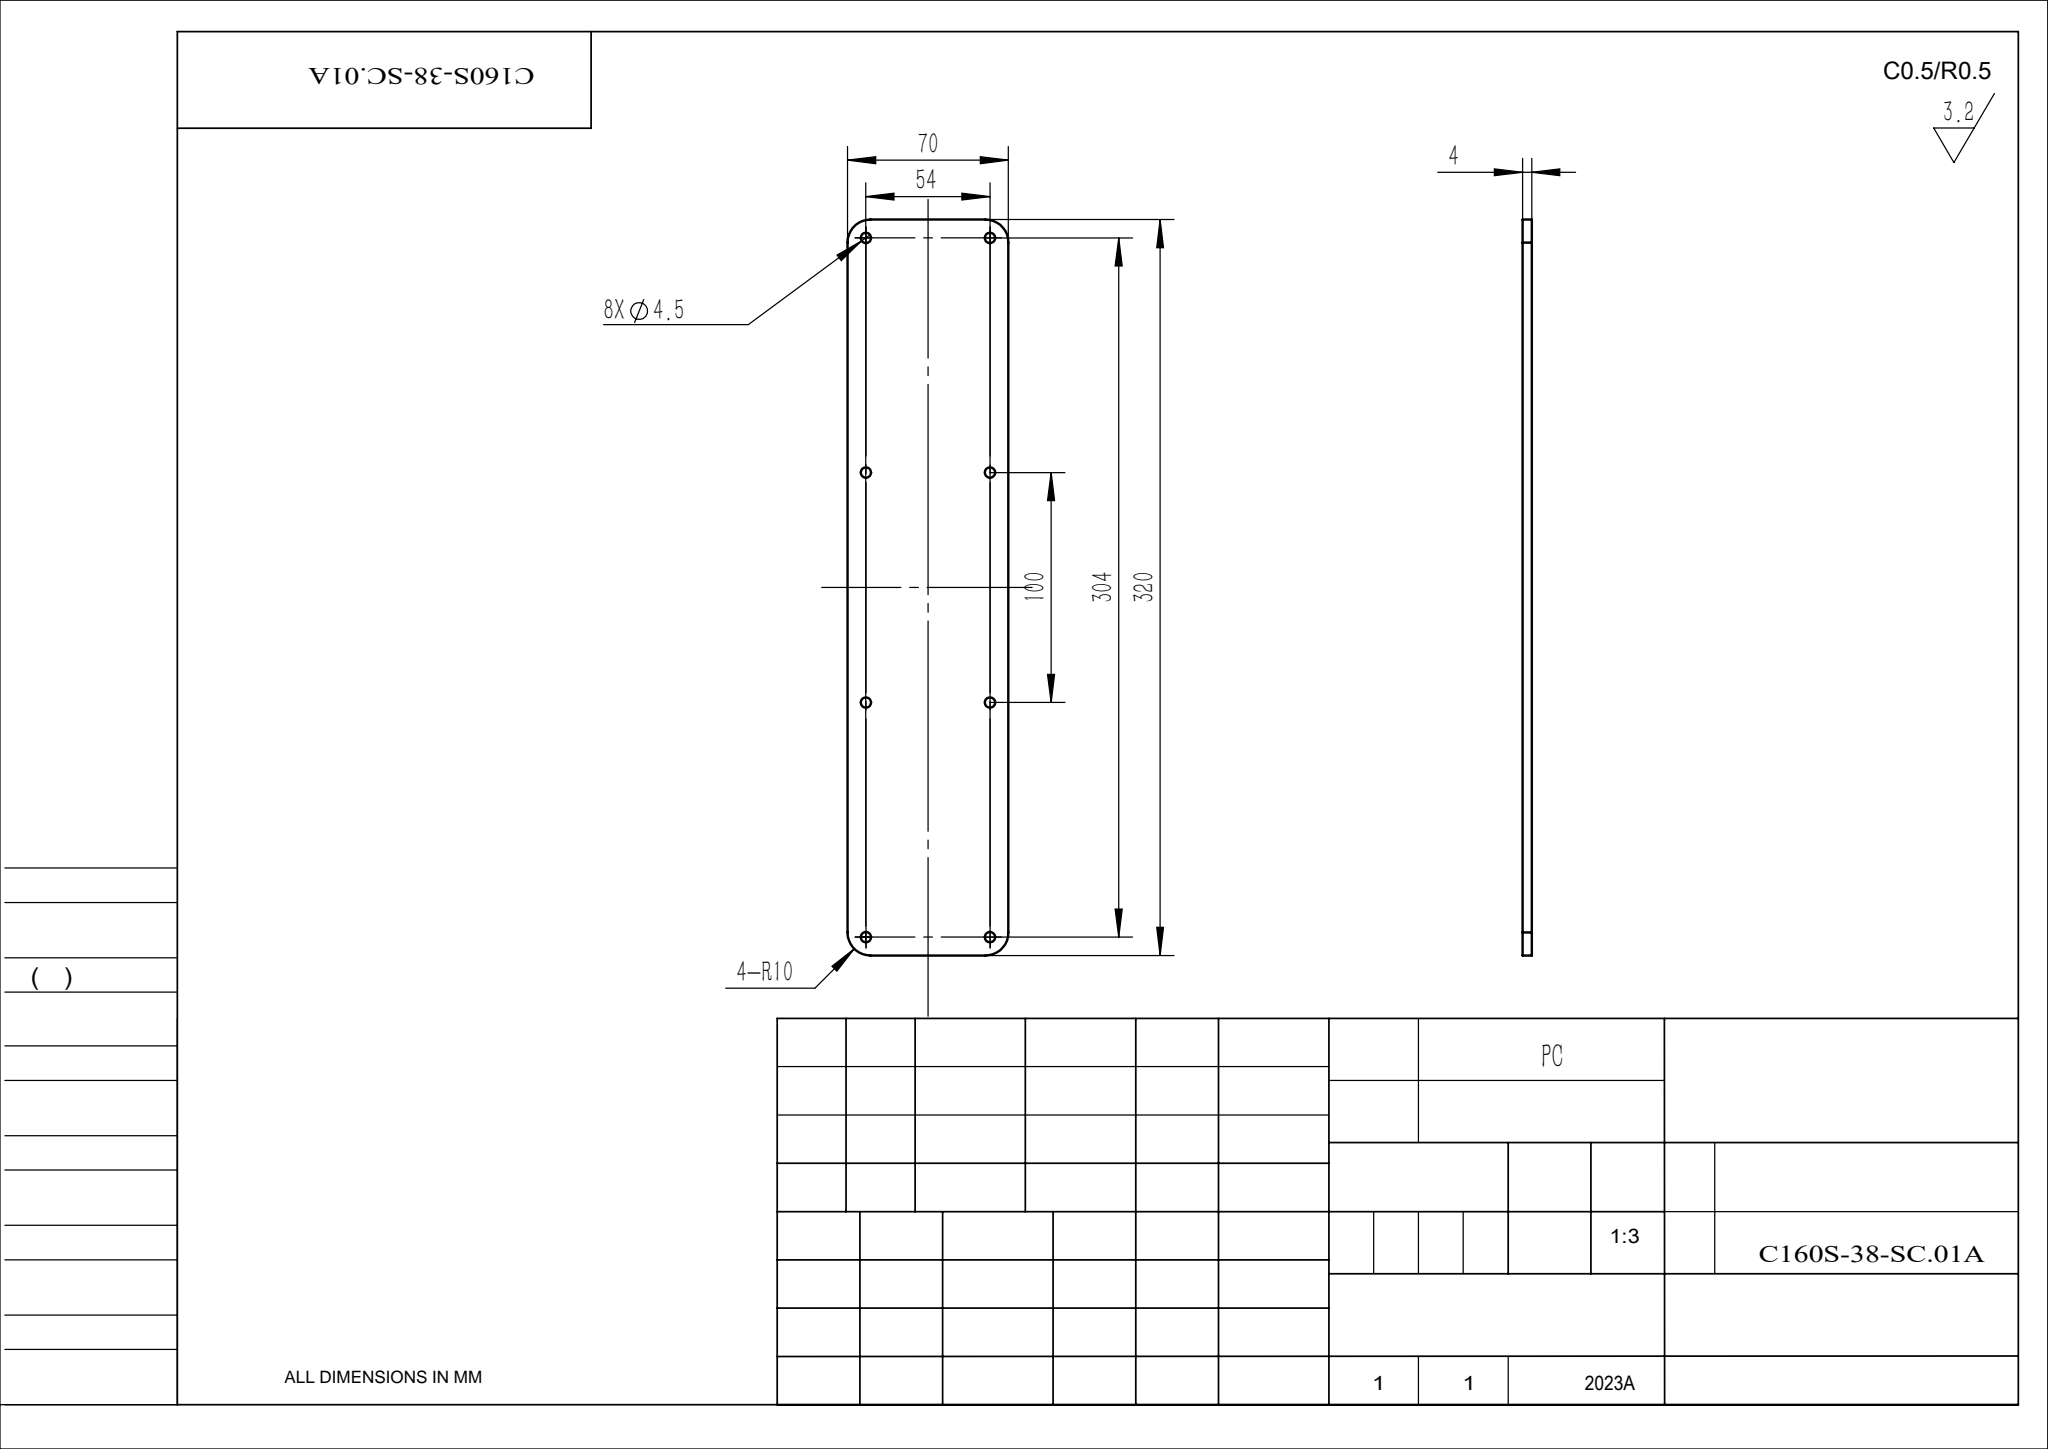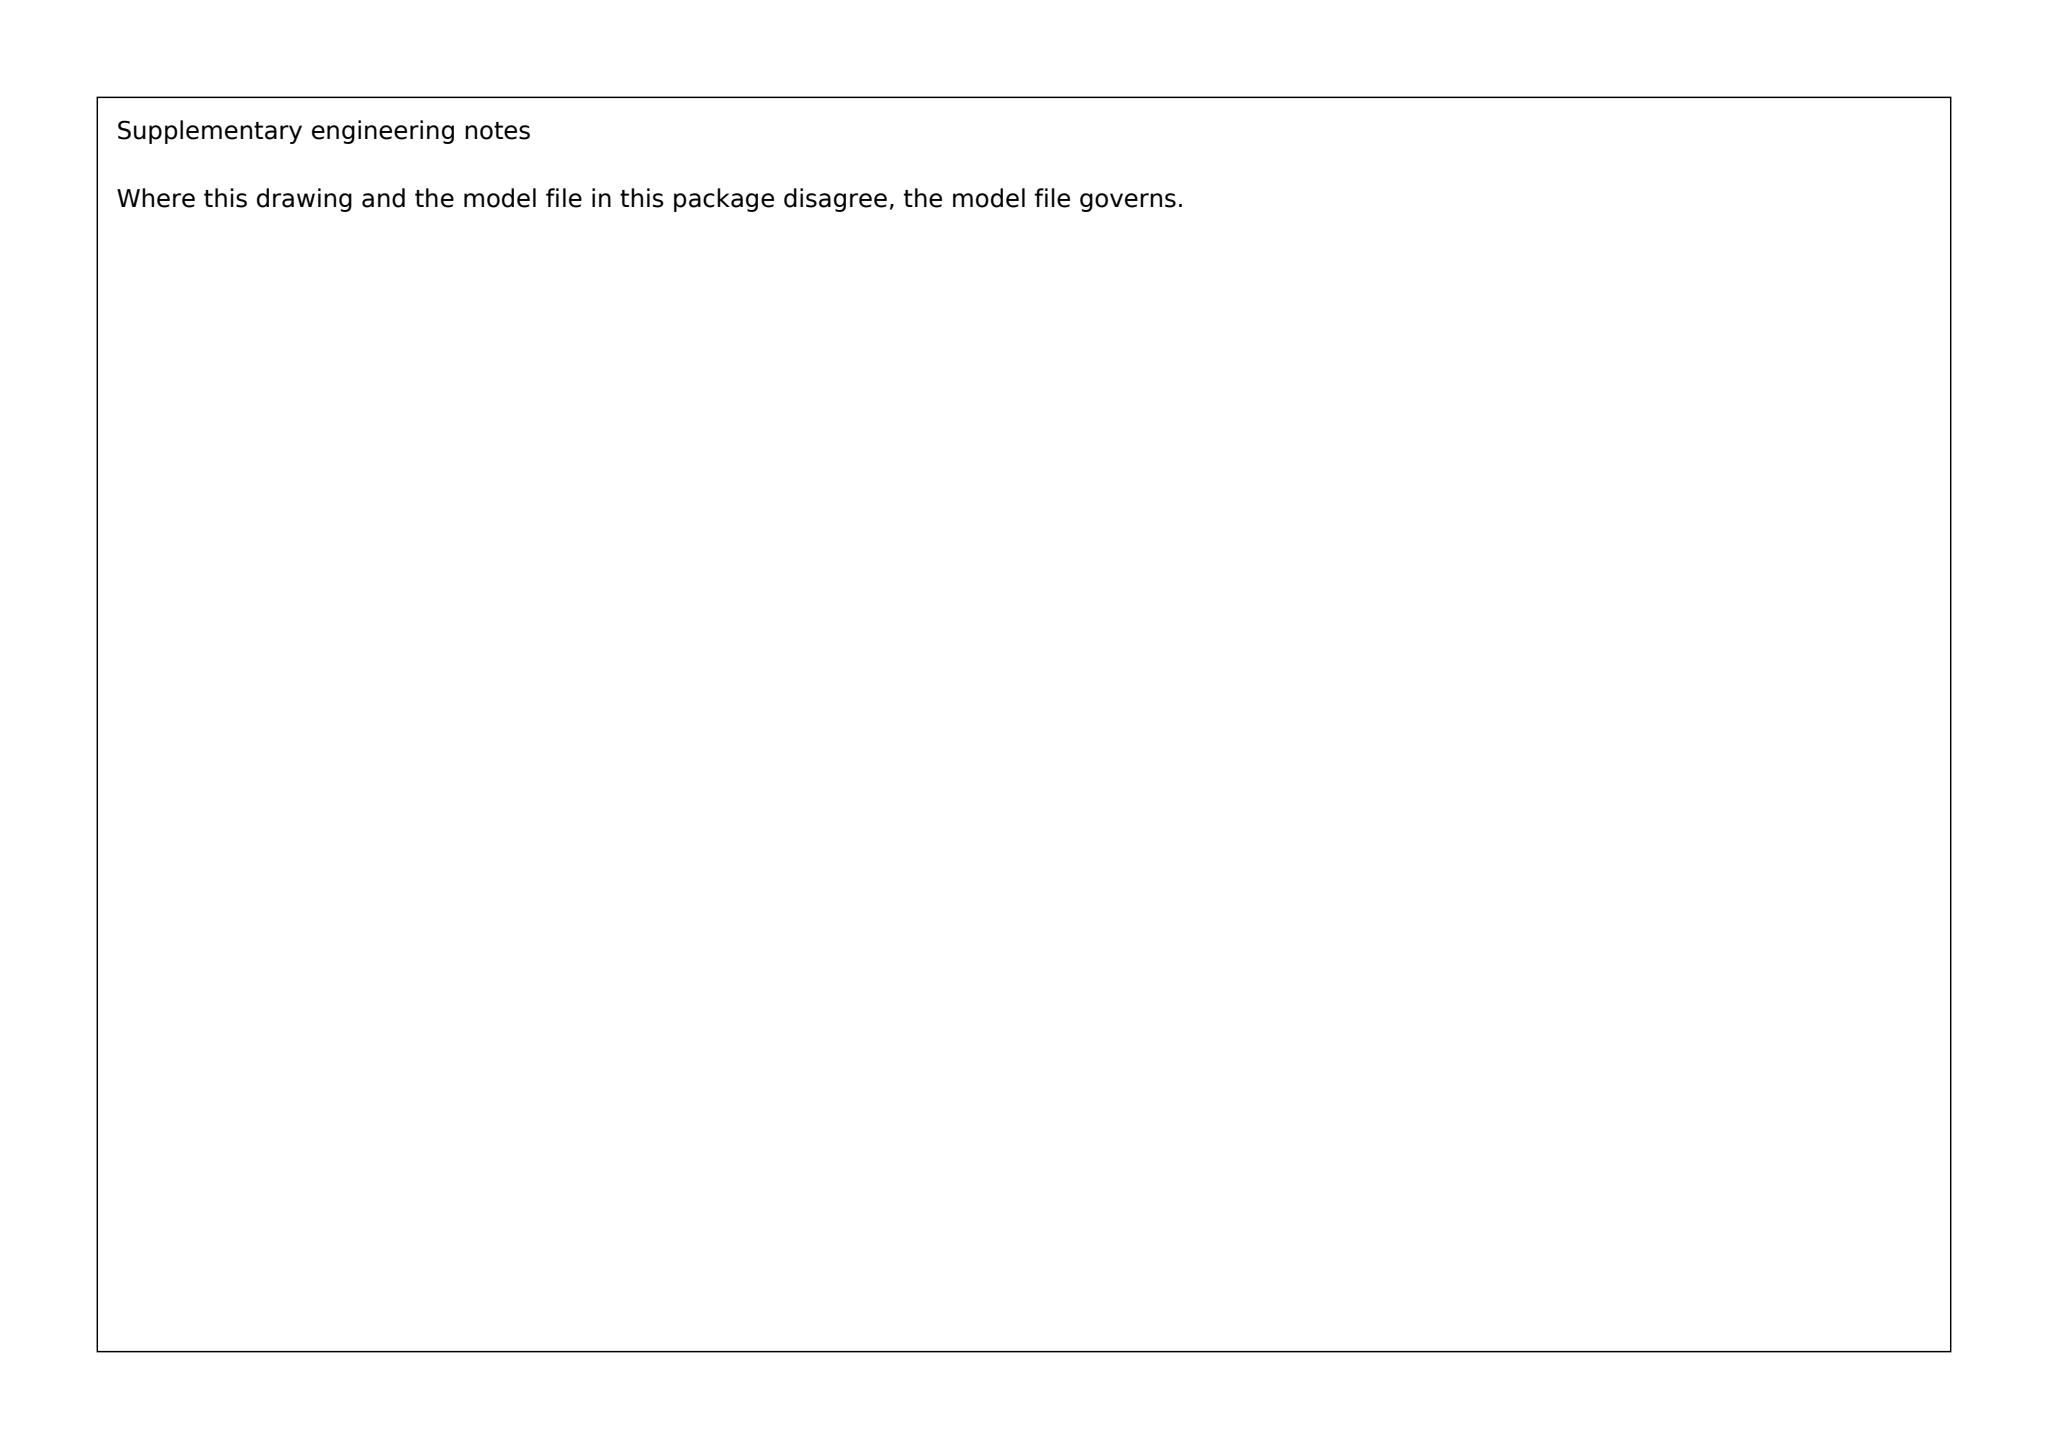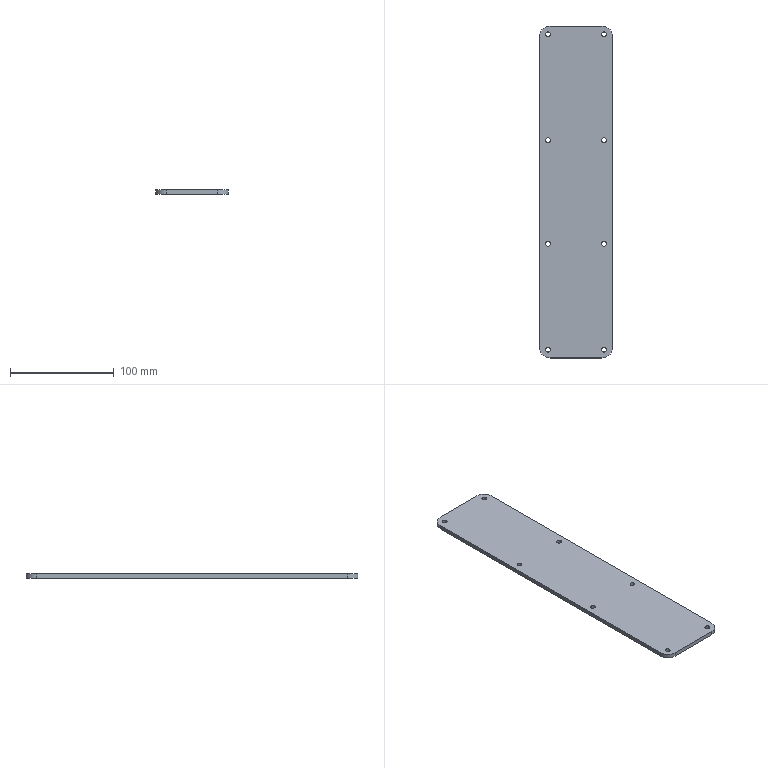Part | SolidWorks | mm | material PC | 1 solid | 26 faces | box 70 x 320 x 4 mm | volume 88748 mm3 | cylinder 20 | plane 6 | commonest cylinder face diameters 4.5 x16 20 x4
build123d program:
from build123d import *

# Parameters (mm, degrees)
SKETCH1_W           = 70
SKETCH1_H           = 320
BOSS_EXTRUDE1_DEPTH = 4
FILLET1_R           = 10
SKETCH2_R           = 2.25
CUT_EXTRUDE1_DEPTH  = 164.832


with BuildPart() as part:
    # Sketch1 → Boss-Extrude1 (new body)
    with BuildSketch(Plane.XY):
        Rectangle(SKETCH1_W, SKETCH1_H)
    extrude(amount=BOSS_EXTRUDE1_DEPTH)

    # Fillet1
    fillet1_edges = [part.edges().sort_by_distance(p)[0] for p in [
        (-35, 160, 2),
        (35, 160, 2),
        (35, -160, 2),
        (-35, -160, 2),
    ]]
    fillet(fillet1_edges, radius=FILLET1_R)

    # Sketch2 → Cut-Extrude1 (cut, through all)
    with BuildSketch(Plane.XY.offset(4)):
        with Locations((27, -152)):
            Circle(SKETCH2_R)
        with Locations((-27, -152)):
            Circle(SKETCH2_R)
        with Locations((27, 152)):
            Circle(SKETCH2_R)
        with Locations((-27, 152)):
            Circle(SKETCH2_R)
        with Locations((-27, 50)):
            Circle(SKETCH2_R)
        with Locations((-27, -50)):
            Circle(SKETCH2_R)
        with Locations((27, 50)):
            Circle(SKETCH2_R)
        with Locations((27, -50)):
            Circle(SKETCH2_R)
    extrude(amount=-CUT_EXTRUDE1_DEPTH, mode=Mode.SUBTRACT)


solid = part.part
STEP:
#1=CARTESIAN_POINT('',(-29.25,50.,0.));
#2=VERTEX_POINT('',#1);
#3=CARTESIAN_POINT('',(-24.75,50.,0.));
#4=VERTEX_POINT('',#3);
#5=CARTESIAN_POINT('',(-27.,50.,0.));
#6=DIRECTION('',(0.,0.,1.));
#7=DIRECTION('',(1.,0.,0.));
#8=AXIS2_PLACEMENT_3D('',#5,#6,#7);
#9=CIRCLE('',#8,2.25);
#10=EDGE_CURVE('',#2,#4,#9,.T.);
#11=ORIENTED_EDGE('',*,*,#10,.F.);
#12=CARTESIAN_POINT('',(-29.25,50.,4.));
#13=VERTEX_POINT('',#12);
#14=CARTESIAN_POINT('',(-29.25,50.,0.));
#15=DIRECTION('',(0.,0.,1.));
#16=VECTOR('',#15,1000.);
#17=LINE('',#14,#16);
#18=EDGE_CURVE('',#2,#13,#17,.T.);
#19=ORIENTED_EDGE('',*,*,#18,.T.);
#20=CARTESIAN_POINT('',(-24.75,50.,4.));
#21=VERTEX_POINT('',#20);
#22=CARTESIAN_POINT('',(-27.,50.,4.));
#23=DIRECTION('',(0.,0.,1.));
#24=DIRECTION('',(1.,0.,0.));
#25=AXIS2_PLACEMENT_3D('',#22,#23,#24);
#26=CIRCLE('',#25,2.25);
#27=EDGE_CURVE('',#13,#21,#26,.T.);
#28=ORIENTED_EDGE('',*,*,#27,.T.);
#29=CARTESIAN_POINT('',(-24.75,50.,0.));
#30=DIRECTION('',(0.,0.,1.));
#31=VECTOR('',#30,1000.);
#32=LINE('',#29,#31);
#33=EDGE_CURVE('',#4,#21,#32,.T.);
#34=ORIENTED_EDGE('',*,*,#33,.F.);
#35=EDGE_LOOP('',(#11,#19,#28,#34));
#36=FACE_OUTER_BOUND('',#35,.T.);
#37=CARTESIAN_POINT('',(-27.,50.,0.));
#38=DIRECTION('',(0.,0.,1.));
#39=DIRECTION('',(1.,0.,0.));
#40=AXIS2_PLACEMENT_3D('',#37,#38,#39);
#41=CYLINDRICAL_SURFACE('',#40,2.25);
#42=ADVANCED_FACE('',(#36),#41,.F.);
#43=CARTESIAN_POINT('',(-29.25,152.,0.));
#44=VERTEX_POINT('',#43);
#45=CARTESIAN_POINT('',(-24.75,152.,0.));
#46=VERTEX_POINT('',#45);
#47=CARTESIAN_POINT('',(-27.,152.,0.));
#48=DIRECTION('',(0.,0.,1.));
#49=DIRECTION('',(1.,0.,0.));
#50=AXIS2_PLACEMENT_3D('',#47,#48,#49);
#51=CIRCLE('',#50,2.25);
#52=EDGE_CURVE('',#44,#46,#51,.T.);
#53=ORIENTED_EDGE('',*,*,#52,.F.);
#54=CARTESIAN_POINT('',(-29.25,152.,4.));
#55=VERTEX_POINT('',#54);
#56=CARTESIAN_POINT('',(-29.25,152.,0.));
#57=DIRECTION('',(0.,0.,1.));
#58=VECTOR('',#57,1000.);
#59=LINE('',#56,#58);
#60=EDGE_CURVE('',#44,#55,#59,.T.);
#61=ORIENTED_EDGE('',*,*,#60,.T.);
#62=CARTESIAN_POINT('',(-24.75,152.,4.));
#63=VERTEX_POINT('',#62);
#64=CARTESIAN_POINT('',(-27.,152.,4.));
#65=DIRECTION('',(0.,0.,1.));
#66=DIRECTION('',(1.,0.,0.));
#67=AXIS2_PLACEMENT_3D('',#64,#65,#66);
#68=CIRCLE('',#67,2.25);
#69=EDGE_CURVE('',#55,#63,#68,.T.);
#70=ORIENTED_EDGE('',*,*,#69,.T.);
#71=CARTESIAN_POINT('',(-24.75,152.,0.));
#72=DIRECTION('',(0.,0.,1.));
#73=VECTOR('',#72,1000.);
#74=LINE('',#71,#73);
#75=EDGE_CURVE('',#46,#63,#74,.T.);
#76=ORIENTED_EDGE('',*,*,#75,.F.);
#77=EDGE_LOOP('',(#53,#61,#70,#76));
#78=FACE_OUTER_BOUND('',#77,.T.);
#79=CARTESIAN_POINT('',(-27.,152.,0.));
#80=DIRECTION('',(0.,0.,1.));
#81=DIRECTION('',(1.,0.,0.));
#82=AXIS2_PLACEMENT_3D('',#79,#80,#81);
#83=CYLINDRICAL_SURFACE('',#82,2.25);
#84=ADVANCED_FACE('',(#78),#83,.F.);
#85=CARTESIAN_POINT('',(24.75,152.,0.));
#86=VERTEX_POINT('',#85);
#87=CARTESIAN_POINT('',(29.25,152.,0.));
#88=VERTEX_POINT('',#87);
#89=CARTESIAN_POINT('',(27.,152.,0.));
#90=DIRECTION('',(0.,0.,1.));
#91=DIRECTION('',(1.,0.,0.));
#92=AXIS2_PLACEMENT_3D('',#89,#90,#91);
#93=CIRCLE('',#92,2.25);
#94=EDGE_CURVE('',#86,#88,#93,.T.);
#95=ORIENTED_EDGE('',*,*,#94,.F.);
#96=CARTESIAN_POINT('',(24.75,152.,4.));
#97=VERTEX_POINT('',#96);
#98=CARTESIAN_POINT('',(24.75,152.,0.));
#99=DIRECTION('',(0.,0.,1.));
#100=VECTOR('',#99,1000.);
#101=LINE('',#98,#100);
#102=EDGE_CURVE('',#86,#97,#101,.T.);
#103=ORIENTED_EDGE('',*,*,#102,.T.);
#104=CARTESIAN_POINT('',(29.25,152.,4.));
#105=VERTEX_POINT('',#104);
#106=CARTESIAN_POINT('',(27.,152.,4.));
#107=DIRECTION('',(0.,0.,1.));
#108=DIRECTION('',(1.,0.,0.));
#109=AXIS2_PLACEMENT_3D('',#106,#107,#108);
#110=CIRCLE('',#109,2.25);
#111=EDGE_CURVE('',#97,#105,#110,.T.);
#112=ORIENTED_EDGE('',*,*,#111,.T.);
#113=CARTESIAN_POINT('',(29.25,152.,0.));
#114=DIRECTION('',(0.,0.,1.));
#115=VECTOR('',#114,1000.);
#116=LINE('',#113,#115);
#117=EDGE_CURVE('',#88,#105,#116,.T.);
#118=ORIENTED_EDGE('',*,*,#117,.F.);
#119=EDGE_LOOP('',(#95,#103,#112,#118));
#120=FACE_OUTER_BOUND('',#119,.T.);
#121=CARTESIAN_POINT('',(27.,152.,0.));
#122=DIRECTION('',(0.,0.,1.));
#123=DIRECTION('',(1.,0.,0.));
#124=AXIS2_PLACEMENT_3D('',#121,#122,#123);
#125=CYLINDRICAL_SURFACE('',#124,2.25);
#126=ADVANCED_FACE('',(#120),#125,.F.);
#127=CARTESIAN_POINT('',(-29.25,-152.,0.));
#128=VERTEX_POINT('',#127);
#129=CARTESIAN_POINT('',(-24.75,-152.,0.));
#130=VERTEX_POINT('',#129);
#131=CARTESIAN_POINT('',(-27.,-152.,0.));
#132=DIRECTION('',(0.,0.,1.));
#133=DIRECTION('',(1.,0.,0.));
#134=AXIS2_PLACEMENT_3D('',#131,#132,#133);
#135=CIRCLE('',#134,2.25);
#136=EDGE_CURVE('',#128,#130,#135,.T.);
#137=ORIENTED_EDGE('',*,*,#136,.F.);
#138=CARTESIAN_POINT('',(-29.25,-152.,4.));
#139=VERTEX_POINT('',#138);
#140=CARTESIAN_POINT('',(-29.25,-152.,0.));
#141=DIRECTION('',(0.,0.,1.));
#142=VECTOR('',#141,1000.);
#143=LINE('',#140,#142);
#144=EDGE_CURVE('',#128,#139,#143,.T.);
#145=ORIENTED_EDGE('',*,*,#144,.T.);
#146=CARTESIAN_POINT('',(-24.75,-152.,4.));
#147=VERTEX_POINT('',#146);
#148=CARTESIAN_POINT('',(-27.,-152.,4.));
#149=DIRECTION('',(0.,0.,1.));
#150=DIRECTION('',(1.,0.,0.));
#151=AXIS2_PLACEMENT_3D('',#148,#149,#150);
#152=CIRCLE('',#151,2.25);
#153=EDGE_CURVE('',#139,#147,#152,.T.);
#154=ORIENTED_EDGE('',*,*,#153,.T.);
#155=CARTESIAN_POINT('',(-24.75,-152.,0.));
#156=DIRECTION('',(0.,0.,1.));
#157=VECTOR('',#156,1000.);
#158=LINE('',#155,#157);
#159=EDGE_CURVE('',#130,#147,#158,.T.);
#160=ORIENTED_EDGE('',*,*,#159,.F.);
#161=EDGE_LOOP('',(#137,#145,#154,#160));
#162=FACE_OUTER_BOUND('',#161,.T.);
#163=CARTESIAN_POINT('',(-27.,-152.,0.));
#164=DIRECTION('',(0.,0.,1.));
#165=DIRECTION('',(1.,0.,0.));
#166=AXIS2_PLACEMENT_3D('',#163,#164,#165);
#167=CYLINDRICAL_SURFACE('',#166,2.25);
#168=ADVANCED_FACE('',(#162),#167,.F.);
#169=CARTESIAN_POINT('',(24.75,-50.,0.));
#170=VERTEX_POINT('',#169);
#171=CARTESIAN_POINT('',(29.25,-50.,0.));
#172=VERTEX_POINT('',#171);
#173=CARTESIAN_POINT('',(27.,-50.,0.));
#174=DIRECTION('',(0.,0.,1.));
#175=DIRECTION('',(1.,0.,0.));
#176=AXIS2_PLACEMENT_3D('',#173,#174,#175);
#177=CIRCLE('',#176,2.25);
#178=EDGE_CURVE('',#170,#172,#177,.T.);
#179=ORIENTED_EDGE('',*,*,#178,.F.);
#180=CARTESIAN_POINT('',(24.75,-50.,4.));
#181=VERTEX_POINT('',#180);
#182=CARTESIAN_POINT('',(24.75,-50.,0.));
#183=DIRECTION('',(0.,0.,1.));
#184=VECTOR('',#183,1000.);
#185=LINE('',#182,#184);
#186=EDGE_CURVE('',#170,#181,#185,.T.);
#187=ORIENTED_EDGE('',*,*,#186,.T.);
#188=CARTESIAN_POINT('',(29.25,-50.,4.));
#189=VERTEX_POINT('',#188);
#190=CARTESIAN_POINT('',(27.,-50.,4.));
#191=DIRECTION('',(0.,0.,1.));
#192=DIRECTION('',(1.,0.,0.));
#193=AXIS2_PLACEMENT_3D('',#190,#191,#192);
#194=CIRCLE('',#193,2.25);
#195=EDGE_CURVE('',#181,#189,#194,.T.);
#196=ORIENTED_EDGE('',*,*,#195,.T.);
#197=CARTESIAN_POINT('',(29.25,-50.,0.));
#198=DIRECTION('',(0.,0.,1.));
#199=VECTOR('',#198,1000.);
#200=LINE('',#197,#199);
#201=EDGE_CURVE('',#172,#189,#200,.T.);
#202=ORIENTED_EDGE('',*,*,#201,.F.);
#203=EDGE_LOOP('',(#179,#187,#196,#202));
#204=FACE_OUTER_BOUND('',#203,.T.);
#205=CARTESIAN_POINT('',(27.,-50.,0.));
#206=DIRECTION('',(0.,0.,1.));
#207=DIRECTION('',(1.,0.,0.));
#208=AXIS2_PLACEMENT_3D('',#205,#206,#207);
#209=CYLINDRICAL_SURFACE('',#208,2.25);
#210=ADVANCED_FACE('',(#204),#209,.F.);
#211=CARTESIAN_POINT('',(24.75,50.,0.));
#212=VERTEX_POINT('',#211);
#213=CARTESIAN_POINT('',(29.25,50.,0.));
#214=VERTEX_POINT('',#213);
#215=CARTESIAN_POINT('',(27.,50.,0.));
#216=DIRECTION('',(0.,0.,1.));
#217=DIRECTION('',(1.,0.,0.));
#218=AXIS2_PLACEMENT_3D('',#215,#216,#217);
#219=CIRCLE('',#218,2.25);
#220=EDGE_CURVE('',#212,#214,#219,.T.);
#221=ORIENTED_EDGE('',*,*,#220,.F.);
#222=CARTESIAN_POINT('',(24.75,50.,4.));
#223=VERTEX_POINT('',#222);
#224=CARTESIAN_POINT('',(24.75,50.,0.));
#225=DIRECTION('',(0.,0.,1.));
#226=VECTOR('',#225,1000.);
#227=LINE('',#224,#226);
#228=EDGE_CURVE('',#212,#223,#227,.T.);
#229=ORIENTED_EDGE('',*,*,#228,.T.);
#230=CARTESIAN_POINT('',(29.25,50.,4.));
#231=VERTEX_POINT('',#230);
#232=CARTESIAN_POINT('',(27.,50.,4.));
#233=DIRECTION('',(0.,0.,1.));
#234=DIRECTION('',(1.,0.,0.));
#235=AXIS2_PLACEMENT_3D('',#232,#233,#234);
#236=CIRCLE('',#235,2.25);
#237=EDGE_CURVE('',#223,#231,#236,.T.);
#238=ORIENTED_EDGE('',*,*,#237,.T.);
#239=CARTESIAN_POINT('',(29.25,50.,0.));
#240=DIRECTION('',(0.,0.,1.));
#241=VECTOR('',#240,1000.);
#242=LINE('',#239,#241);
#243=EDGE_CURVE('',#214,#231,#242,.T.);
#244=ORIENTED_EDGE('',*,*,#243,.F.);
#245=EDGE_LOOP('',(#221,#229,#238,#244));
#246=FACE_OUTER_BOUND('',#245,.T.);
#247=CARTESIAN_POINT('',(27.,50.,0.));
#248=DIRECTION('',(0.,0.,1.));
#249=DIRECTION('',(1.,0.,0.));
#250=AXIS2_PLACEMENT_3D('',#247,#248,#249);
#251=CYLINDRICAL_SURFACE('',#250,2.25);
#252=ADVANCED_FACE('',(#246),#251,.F.);
#253=CARTESIAN_POINT('',(-29.25,-50.,0.));
#254=VERTEX_POINT('',#253);
#255=CARTESIAN_POINT('',(-24.75,-50.,0.));
#256=VERTEX_POINT('',#255);
#257=CARTESIAN_POINT('',(-27.,-50.,0.));
#258=DIRECTION('',(0.,0.,1.));
#259=DIRECTION('',(1.,0.,0.));
#260=AXIS2_PLACEMENT_3D('',#257,#258,#259);
#261=CIRCLE('',#260,2.25);
#262=EDGE_CURVE('',#254,#256,#261,.T.);
#263=ORIENTED_EDGE('',*,*,#262,.F.);
#264=CARTESIAN_POINT('',(-29.25,-50.,4.));
#265=VERTEX_POINT('',#264);
#266=CARTESIAN_POINT('',(-29.25,-50.,0.));
#267=DIRECTION('',(0.,0.,1.));
#268=VECTOR('',#267,1000.);
#269=LINE('',#266,#268);
#270=EDGE_CURVE('',#254,#265,#269,.T.);
#271=ORIENTED_EDGE('',*,*,#270,.T.);
#272=CARTESIAN_POINT('',(-24.75,-50.,4.));
#273=VERTEX_POINT('',#272);
#274=CARTESIAN_POINT('',(-27.,-50.,4.));
#275=DIRECTION('',(0.,0.,1.));
#276=DIRECTION('',(1.,0.,0.));
#277=AXIS2_PLACEMENT_3D('',#274,#275,#276);
#278=CIRCLE('',#277,2.25);
#279=EDGE_CURVE('',#265,#273,#278,.T.);
#280=ORIENTED_EDGE('',*,*,#279,.T.);
#281=CARTESIAN_POINT('',(-24.75,-50.,0.));
#282=DIRECTION('',(0.,0.,1.));
#283=VECTOR('',#282,1000.);
#284=LINE('',#281,#283);
#285=EDGE_CURVE('',#256,#273,#284,.T.);
#286=ORIENTED_EDGE('',*,*,#285,.F.);
#287=EDGE_LOOP('',(#263,#271,#280,#286));
#288=FACE_OUTER_BOUND('',#287,.T.);
#289=CARTESIAN_POINT('',(-27.,-50.,0.));
#290=DIRECTION('',(0.,0.,1.));
#291=DIRECTION('',(1.,0.,0.));
#292=AXIS2_PLACEMENT_3D('',#289,#290,#291);
#293=CYLINDRICAL_SURFACE('',#292,2.25);
#294=ADVANCED_FACE('',(#288),#293,.F.);
#295=CARTESIAN_POINT('',(24.75,-152.,0.));
#296=VERTEX_POINT('',#295);
#297=CARTESIAN_POINT('',(29.25,-152.,0.));
#298=VERTEX_POINT('',#297);
#299=CARTESIAN_POINT('',(27.,-152.,0.));
#300=DIRECTION('',(0.,0.,1.));
#301=DIRECTION('',(1.,0.,0.));
#302=AXIS2_PLACEMENT_3D('',#299,#300,#301);
#303=CIRCLE('',#302,2.25);
#304=EDGE_CURVE('',#296,#298,#303,.T.);
#305=ORIENTED_EDGE('',*,*,#304,.F.);
#306=CARTESIAN_POINT('',(24.75,-152.,4.));
#307=VERTEX_POINT('',#306);
#308=CARTESIAN_POINT('',(24.75,-152.,0.));
#309=DIRECTION('',(0.,0.,1.));
#310=VECTOR('',#309,1000.);
#311=LINE('',#308,#310);
#312=EDGE_CURVE('',#296,#307,#311,.T.);
#313=ORIENTED_EDGE('',*,*,#312,.T.);
#314=CARTESIAN_POINT('',(29.25,-152.,4.));
#315=VERTEX_POINT('',#314);
#316=CARTESIAN_POINT('',(27.,-152.,4.));
#317=DIRECTION('',(0.,0.,1.));
#318=DIRECTION('',(1.,0.,0.));
#319=AXIS2_PLACEMENT_3D('',#316,#317,#318);
#320=CIRCLE('',#319,2.25);
#321=EDGE_CURVE('',#307,#315,#320,.T.);
#322=ORIENTED_EDGE('',*,*,#321,.T.);
#323=CARTESIAN_POINT('',(29.25,-152.,0.));
#324=DIRECTION('',(0.,0.,1.));
#325=VECTOR('',#324,1000.);
#326=LINE('',#323,#325);
#327=EDGE_CURVE('',#298,#315,#326,.T.);
#328=ORIENTED_EDGE('',*,*,#327,.F.);
#329=EDGE_LOOP('',(#305,#313,#322,#328));
#330=FACE_OUTER_BOUND('',#329,.T.);
#331=CARTESIAN_POINT('',(27.,-152.,0.));
#332=DIRECTION('',(0.,0.,1.));
#333=DIRECTION('',(1.,0.,0.));
#334=AXIS2_PLACEMENT_3D('',#331,#332,#333);
#335=CYLINDRICAL_SURFACE('',#334,2.25);
#336=ADVANCED_FACE('',(#330),#335,.F.);
#337=CARTESIAN_POINT('',(-35.,150.,0.));
#338=VERTEX_POINT('',#337);
#339=CARTESIAN_POINT('',(-35.,-150.,0.));
#340=VERTEX_POINT('',#339);
#341=CARTESIAN_POINT('',(-35.,-160.,0.));
#342=DIRECTION('',(0.,-1.,0.));
#343=VECTOR('',#342,1000.);
#344=LINE('',#341,#343);
#345=EDGE_CURVE('',#338,#340,#344,.T.);
#346=ORIENTED_EDGE('',*,*,#345,.T.);
#347=CARTESIAN_POINT('',(-35.,-150.,4.));
#348=VERTEX_POINT('',#347);
#349=CARTESIAN_POINT('',(-35.,-150.,4.));
#350=DIRECTION('',(0.,0.,1.));
#351=VECTOR('',#350,1000.);
#352=LINE('',#349,#351);
#353=EDGE_CURVE('',#340,#348,#352,.T.);
#354=ORIENTED_EDGE('',*,*,#353,.T.);
#355=CARTESIAN_POINT('',(-35.,150.,4.));
#356=VERTEX_POINT('',#355);
#357=CARTESIAN_POINT('',(-35.,-160.,4.));
#358=DIRECTION('',(0.,-1.,0.));
#359=VECTOR('',#358,1000.);
#360=LINE('',#357,#359);
#361=EDGE_CURVE('',#356,#348,#360,.T.);
#362=ORIENTED_EDGE('',*,*,#361,.F.);
#363=CARTESIAN_POINT('',(-35.,150.,4.));
#364=DIRECTION('',(0.,0.,-1.));
#365=VECTOR('',#364,1000.);
#366=LINE('',#363,#365);
#367=EDGE_CURVE('',#356,#338,#366,.T.);
#368=ORIENTED_EDGE('',*,*,#367,.T.);
#369=EDGE_LOOP('',(#346,#354,#362,#368));
#370=FACE_OUTER_BOUND('',#369,.T.);
#371=CARTESIAN_POINT('',(-35.,-160.,4.));
#372=DIRECTION('',(1.,0.,0.));
#373=DIRECTION('',(0.,0.,-1.));
#374=AXIS2_PLACEMENT_3D('',#371,#372,#373);
#375=PLANE('',#374);
#376=ADVANCED_FACE('',(#370),#375,.F.);
#377=CARTESIAN_POINT('',(-25.,-160.,4.));
#378=VERTEX_POINT('',#377);
#379=CARTESIAN_POINT('',(25.,-160.,4.));
#380=VERTEX_POINT('',#379);
#381=CARTESIAN_POINT('',(35.,-160.,4.));
#382=DIRECTION('',(1.,0.,0.));
#383=VECTOR('',#382,1000.);
#384=LINE('',#381,#383);
#385=EDGE_CURVE('',#378,#380,#384,.T.);
#386=ORIENTED_EDGE('',*,*,#385,.F.);
#387=CARTESIAN_POINT('',(-25.,-160.,0.));
#388=VERTEX_POINT('',#387);
#389=CARTESIAN_POINT('',(-25.,-160.,4.));
#390=DIRECTION('',(0.,0.,-1.));
#391=VECTOR('',#390,1000.);
#392=LINE('',#389,#391);
#393=EDGE_CURVE('',#378,#388,#392,.T.);
#394=ORIENTED_EDGE('',*,*,#393,.T.);
#395=CARTESIAN_POINT('',(25.,-160.,0.));
#396=VERTEX_POINT('',#395);
#397=CARTESIAN_POINT('',(35.,-160.,0.));
#398=DIRECTION('',(1.,0.,0.));
#399=VECTOR('',#398,1000.);
#400=LINE('',#397,#399);
#401=EDGE_CURVE('',#388,#396,#400,.T.);
#402=ORIENTED_EDGE('',*,*,#401,.T.);
#403=CARTESIAN_POINT('',(25.,-160.,4.));
#404=DIRECTION('',(0.,0.,1.));
#405=VECTOR('',#404,1000.);
#406=LINE('',#403,#405);
#407=EDGE_CURVE('',#396,#380,#406,.T.);
#408=ORIENTED_EDGE('',*,*,#407,.T.);
#409=EDGE_LOOP('',(#386,#394,#402,#408));
#410=FACE_OUTER_BOUND('',#409,.T.);
#411=CARTESIAN_POINT('',(35.,-160.,4.));
#412=DIRECTION('',(0.,1.,0.));
#413=DIRECTION('',(0.,0.,1.));
#414=AXIS2_PLACEMENT_3D('',#411,#412,#413);
#415=PLANE('',#414);
#416=ADVANCED_FACE('',(#410),#415,.F.);
#417=CARTESIAN_POINT('',(35.,-150.,4.));
#418=VERTEX_POINT('',#417);
#419=CARTESIAN_POINT('',(35.,150.,4.));
#420=VERTEX_POINT('',#419);
#421=CARTESIAN_POINT('',(35.,-160.,4.));
#422=DIRECTION('',(0.,1.,0.));
#423=VECTOR('',#422,1000.);
#424=LINE('',#421,#423);
#425=EDGE_CURVE('',#418,#420,#424,.T.);
#426=ORIENTED_EDGE('',*,*,#425,.F.);
#427=CARTESIAN_POINT('',(35.,-150.,0.));
#428=VERTEX_POINT('',#427);
#429=CARTESIAN_POINT('',(35.,-150.,4.));
#430=DIRECTION('',(0.,0.,-1.));
#431=VECTOR('',#430,1000.);
#432=LINE('',#429,#431);
#433=EDGE_CURVE('',#418,#428,#432,.T.);
#434=ORIENTED_EDGE('',*,*,#433,.T.);
#435=CARTESIAN_POINT('',(35.,150.,0.));
#436=VERTEX_POINT('',#435);
#437=CARTESIAN_POINT('',(35.,-160.,0.));
#438=DIRECTION('',(0.,1.,0.));
#439=VECTOR('',#438,1000.);
#440=LINE('',#437,#439);
#441=EDGE_CURVE('',#428,#436,#440,.T.);
#442=ORIENTED_EDGE('',*,*,#441,.T.);
#443=CARTESIAN_POINT('',(35.,150.,4.));
#444=DIRECTION('',(0.,0.,1.));
#445=VECTOR('',#444,1000.);
#446=LINE('',#443,#445);
#447=EDGE_CURVE('',#436,#420,#446,.T.);
#448=ORIENTED_EDGE('',*,*,#447,.T.);
#449=EDGE_LOOP('',(#426,#434,#442,#448));
#450=FACE_OUTER_BOUND('',#449,.T.);
#451=CARTESIAN_POINT('',(35.,-160.,4.));
#452=DIRECTION('',(-1.,0.,0.));
#453=DIRECTION('',(0.,0.,1.));
#454=AXIS2_PLACEMENT_3D('',#451,#452,#453);
#455=PLANE('',#454);
#456=ADVANCED_FACE('',(#450),#455,.F.);
#457=CARTESIAN_POINT('',(25.,160.,4.));
#458=VERTEX_POINT('',#457);
#459=CARTESIAN_POINT('',(-25.,160.,4.));
#460=VERTEX_POINT('',#459);
#461=CARTESIAN_POINT('',(35.,160.,4.));
#462=DIRECTION('',(-1.,-0.,0.));
#463=VECTOR('',#462,1000.);
#464=LINE('',#461,#463);
#465=EDGE_CURVE('',#458,#460,#464,.T.);
#466=ORIENTED_EDGE('',*,*,#465,.F.);
#467=CARTESIAN_POINT('',(25.,160.,0.));
#468=VERTEX_POINT('',#467);
#469=CARTESIAN_POINT('',(25.,160.,4.));
#470=DIRECTION('',(0.,0.,-1.));
#471=VECTOR('',#470,1000.);
#472=LINE('',#469,#471);
#473=EDGE_CURVE('',#458,#468,#472,.T.);
#474=ORIENTED_EDGE('',*,*,#473,.T.);
#475=CARTESIAN_POINT('',(-25.,160.,0.));
#476=VERTEX_POINT('',#475);
#477=CARTESIAN_POINT('',(35.,160.,0.));
#478=DIRECTION('',(-1.,-0.,0.));
#479=VECTOR('',#478,1000.);
#480=LINE('',#477,#479);
#481=EDGE_CURVE('',#468,#476,#480,.T.);
#482=ORIENTED_EDGE('',*,*,#481,.T.);
#483=CARTESIAN_POINT('',(-25.,160.,4.));
#484=DIRECTION('',(0.,0.,1.));
#485=VECTOR('',#484,1000.);
#486=LINE('',#483,#485);
#487=EDGE_CURVE('',#476,#460,#486,.T.);
#488=ORIENTED_EDGE('',*,*,#487,.T.);
#489=EDGE_LOOP('',(#466,#474,#482,#488));
#490=FACE_OUTER_BOUND('',#489,.T.);
#491=CARTESIAN_POINT('',(35.,160.,4.));
#492=DIRECTION('',(0.,-1.,0.));
#493=DIRECTION('',(1.,0.,0.));
#494=AXIS2_PLACEMENT_3D('',#491,#492,#493);
#495=PLANE('',#494);
#496=ADVANCED_FACE('',(#490),#495,.F.);
#497=CARTESIAN_POINT('',(-27.,50.,4.));
#498=DIRECTION('',(0.,0.,1.));
#499=DIRECTION('',(1.,0.,0.));
#500=AXIS2_PLACEMENT_3D('',#497,#498,#499);
#501=CIRCLE('',#500,2.25);
#502=EDGE_CURVE('',#21,#13,#501,.T.);
#503=ORIENTED_EDGE('',*,*,#502,.F.);
#504=ORIENTED_EDGE('',*,*,#27,.F.);
#505=EDGE_LOOP('',(#503,#504));
#506=FACE_BOUND('',#505,.T.);
#507=CARTESIAN_POINT('',(-27.,152.,4.));
#508=DIRECTION('',(0.,0.,1.));
#509=DIRECTION('',(1.,0.,0.));
#510=AXIS2_PLACEMENT_3D('',#507,#508,#509);
#511=CIRCLE('',#510,2.25);
#512=EDGE_CURVE('',#63,#55,#511,.T.);
#513=ORIENTED_EDGE('',*,*,#512,.F.);
#514=ORIENTED_EDGE('',*,*,#69,.F.);
#515=EDGE_LOOP('',(#513,#514));
#516=FACE_BOUND('',#515,.T.);
#517=CARTESIAN_POINT('',(27.,152.,4.));
#518=DIRECTION('',(0.,0.,1.));
#519=DIRECTION('',(1.,0.,0.));
#520=AXIS2_PLACEMENT_3D('',#517,#518,#519);
#521=CIRCLE('',#520,2.25);
#522=EDGE_CURVE('',#105,#97,#521,.T.);
#523=ORIENTED_EDGE('',*,*,#522,.F.);
#524=ORIENTED_EDGE('',*,*,#111,.F.);
#525=EDGE_LOOP('',(#523,#524));
#526=FACE_BOUND('',#525,.T.);
#527=CARTESIAN_POINT('',(-27.,-152.,4.));
#528=DIRECTION('',(0.,0.,1.));
#529=DIRECTION('',(1.,0.,0.));
#530=AXIS2_PLACEMENT_3D('',#527,#528,#529);
#531=CIRCLE('',#530,2.25);
#532=EDGE_CURVE('',#147,#139,#531,.T.);
#533=ORIENTED_EDGE('',*,*,#532,.F.);
#534=ORIENTED_EDGE('',*,*,#153,.F.);
#535=EDGE_LOOP('',(#533,#534));
#536=FACE_BOUND('',#535,.T.);
#537=CARTESIAN_POINT('',(27.,-50.,4.));
#538=DIRECTION('',(0.,0.,1.));
#539=DIRECTION('',(1.,0.,0.));
#540=AXIS2_PLACEMENT_3D('',#537,#538,#539);
#541=CIRCLE('',#540,2.25);
#542=EDGE_CURVE('',#189,#181,#541,.T.);
#543=ORIENTED_EDGE('',*,*,#542,.F.);
#544=ORIENTED_EDGE('',*,*,#195,.F.);
#545=EDGE_LOOP('',(#543,#544));
#546=FACE_BOUND('',#545,.T.);
#547=CARTESIAN_POINT('',(27.,50.,4.));
#548=DIRECTION('',(0.,0.,1.));
#549=DIRECTION('',(1.,0.,0.));
#550=AXIS2_PLACEMENT_3D('',#547,#548,#549);
#551=CIRCLE('',#550,2.25);
#552=EDGE_CURVE('',#231,#223,#551,.T.);
#553=ORIENTED_EDGE('',*,*,#552,.F.);
#554=ORIENTED_EDGE('',*,*,#237,.F.);
#555=EDGE_LOOP('',(#553,#554));
#556=FACE_BOUND('',#555,.T.);
#557=CARTESIAN_POINT('',(-27.,-50.,4.));
#558=DIRECTION('',(0.,0.,1.));
#559=DIRECTION('',(1.,0.,0.));
#560=AXIS2_PLACEMENT_3D('',#557,#558,#559);
#561=CIRCLE('',#560,2.25);
#562=EDGE_CURVE('',#273,#265,#561,.T.);
#563=ORIENTED_EDGE('',*,*,#562,.F.);
#564=ORIENTED_EDGE('',*,*,#279,.F.);
#565=EDGE_LOOP('',(#563,#564));
#566=FACE_BOUND('',#565,.T.);
#567=CARTESIAN_POINT('',(27.,-152.,4.));
#568=DIRECTION('',(0.,0.,1.));
#569=DIRECTION('',(1.,0.,0.));
#570=AXIS2_PLACEMENT_3D('',#567,#568,#569);
#571=CIRCLE('',#570,2.25);
#572=EDGE_CURVE('',#315,#307,#571,.T.);
#573=ORIENTED_EDGE('',*,*,#572,.F.);
#574=ORIENTED_EDGE('',*,*,#321,.F.);
#575=EDGE_LOOP('',(#573,#574));
#576=FACE_BOUND('',#575,.T.);
#577=ORIENTED_EDGE('',*,*,#361,.T.);
#578=CARTESIAN_POINT('',(-25.,-150.,4.));
#579=DIRECTION('',(0.,0.,1.));
#580=DIRECTION('',(1.,0.,0.));
#581=AXIS2_PLACEMENT_3D('',#578,#579,#580);
#582=CIRCLE('',#581,10.);
#583=EDGE_CURVE('',#348,#378,#582,.T.);
#584=ORIENTED_EDGE('',*,*,#583,.T.);
#585=ORIENTED_EDGE('',*,*,#385,.T.);
#586=CARTESIAN_POINT('',(25.,-150.,4.));
#587=DIRECTION('',(0.,0.,1.));
#588=DIRECTION('',(1.,0.,0.));
#589=AXIS2_PLACEMENT_3D('',#586,#587,#588);
#590=CIRCLE('',#589,10.);
#591=EDGE_CURVE('',#380,#418,#590,.T.);
#592=ORIENTED_EDGE('',*,*,#591,.T.);
#593=ORIENTED_EDGE('',*,*,#425,.T.);
#594=CARTESIAN_POINT('',(25.,150.,4.));
#595=DIRECTION('',(0.,0.,1.));
#596=DIRECTION('',(1.,0.,0.));
#597=AXIS2_PLACEMENT_3D('',#594,#595,#596);
#598=CIRCLE('',#597,10.);
#599=EDGE_CURVE('',#420,#458,#598,.T.);
#600=ORIENTED_EDGE('',*,*,#599,.T.);
#601=ORIENTED_EDGE('',*,*,#465,.T.);
#602=CARTESIAN_POINT('',(-25.,150.,4.));
#603=DIRECTION('',(0.,0.,1.));
#604=DIRECTION('',(1.,0.,0.));
#605=AXIS2_PLACEMENT_3D('',#602,#603,#604);
#606=CIRCLE('',#605,10.);
#607=EDGE_CURVE('',#460,#356,#606,.T.);
#608=ORIENTED_EDGE('',*,*,#607,.T.);
#609=EDGE_LOOP('',(#577,#584,#585,#592,#593,#600,#601,#608));
#610=FACE_OUTER_BOUND('',#609,.T.);
#611=CARTESIAN_POINT('',(0.,0.,4.));
#612=DIRECTION('',(0.,0.,1.));
#613=DIRECTION('',(1.,0.,0.));
#614=AXIS2_PLACEMENT_3D('',#611,#612,#613);
#615=PLANE('',#614);
#616=ADVANCED_FACE('',(#506,#516,#526,#536,#546,#556,#566,#576,#610),#615,.T.);
#617=CARTESIAN_POINT('',(-27.,50.,0.));
#618=DIRECTION('',(0.,0.,1.));
#619=DIRECTION('',(1.,0.,0.));
#620=AXIS2_PLACEMENT_3D('',#617,#618,#619);
#621=CIRCLE('',#620,2.25);
#622=EDGE_CURVE('',#4,#2,#621,.T.);
#623=ORIENTED_EDGE('',*,*,#622,.T.);
#624=ORIENTED_EDGE('',*,*,#10,.T.);
#625=EDGE_LOOP('',(#623,#624));
#626=FACE_BOUND('',#625,.T.);
#627=CARTESIAN_POINT('',(-27.,152.,0.));
#628=DIRECTION('',(0.,0.,1.));
#629=DIRECTION('',(1.,0.,0.));
#630=AXIS2_PLACEMENT_3D('',#627,#628,#629);
#631=CIRCLE('',#630,2.25);
#632=EDGE_CURVE('',#46,#44,#631,.T.);
#633=ORIENTED_EDGE('',*,*,#632,.T.);
#634=ORIENTED_EDGE('',*,*,#52,.T.);
#635=EDGE_LOOP('',(#633,#634));
#636=FACE_BOUND('',#635,.T.);
#637=CARTESIAN_POINT('',(27.,152.,0.));
#638=DIRECTION('',(0.,0.,1.));
#639=DIRECTION('',(1.,0.,0.));
#640=AXIS2_PLACEMENT_3D('',#637,#638,#639);
#641=CIRCLE('',#640,2.25);
#642=EDGE_CURVE('',#88,#86,#641,.T.);
#643=ORIENTED_EDGE('',*,*,#642,.T.);
#644=ORIENTED_EDGE('',*,*,#94,.T.);
#645=EDGE_LOOP('',(#643,#644));
#646=FACE_BOUND('',#645,.T.);
#647=CARTESIAN_POINT('',(-27.,-152.,0.));
#648=DIRECTION('',(0.,0.,1.));
#649=DIRECTION('',(1.,0.,0.));
#650=AXIS2_PLACEMENT_3D('',#647,#648,#649);
#651=CIRCLE('',#650,2.25);
#652=EDGE_CURVE('',#130,#128,#651,.T.);
#653=ORIENTED_EDGE('',*,*,#652,.T.);
#654=ORIENTED_EDGE('',*,*,#136,.T.);
#655=EDGE_LOOP('',(#653,#654));
#656=FACE_BOUND('',#655,.T.);
#657=CARTESIAN_POINT('',(27.,-50.,0.));
#658=DIRECTION('',(0.,0.,1.));
#659=DIRECTION('',(1.,0.,0.));
#660=AXIS2_PLACEMENT_3D('',#657,#658,#659);
#661=CIRCLE('',#660,2.25);
#662=EDGE_CURVE('',#172,#170,#661,.T.);
#663=ORIENTED_EDGE('',*,*,#662,.T.);
#664=ORIENTED_EDGE('',*,*,#178,.T.);
#665=EDGE_LOOP('',(#663,#664));
#666=FACE_BOUND('',#665,.T.);
#667=CARTESIAN_POINT('',(27.,50.,0.));
#668=DIRECTION('',(0.,0.,1.));
#669=DIRECTION('',(1.,0.,0.));
#670=AXIS2_PLACEMENT_3D('',#667,#668,#669);
#671=CIRCLE('',#670,2.25);
#672=EDGE_CURVE('',#214,#212,#671,.T.);
#673=ORIENTED_EDGE('',*,*,#672,.T.);
#674=ORIENTED_EDGE('',*,*,#220,.T.);
#675=EDGE_LOOP('',(#673,#674));
#676=FACE_BOUND('',#675,.T.);
#677=CARTESIAN_POINT('',(-27.,-50.,0.));
#678=DIRECTION('',(0.,0.,1.));
#679=DIRECTION('',(1.,0.,0.));
#680=AXIS2_PLACEMENT_3D('',#677,#678,#679);
#681=CIRCLE('',#680,2.25);
#682=EDGE_CURVE('',#256,#254,#681,.T.);
#683=ORIENTED_EDGE('',*,*,#682,.T.);
#684=ORIENTED_EDGE('',*,*,#262,.T.);
#685=EDGE_LOOP('',(#683,#684));
#686=FACE_BOUND('',#685,.T.);
#687=CARTESIAN_POINT('',(27.,-152.,0.));
#688=DIRECTION('',(0.,0.,1.));
#689=DIRECTION('',(1.,0.,0.));
#690=AXIS2_PLACEMENT_3D('',#687,#688,#689);
#691=CIRCLE('',#690,2.25);
#692=EDGE_CURVE('',#298,#296,#691,.T.);
#693=ORIENTED_EDGE('',*,*,#692,.T.);
#694=ORIENTED_EDGE('',*,*,#304,.T.);
#695=EDGE_LOOP('',(#693,#694));
#696=FACE_BOUND('',#695,.T.);
#697=ORIENTED_EDGE('',*,*,#401,.F.);
#698=CARTESIAN_POINT('',(-25.,-150.,0.));
#699=DIRECTION('',(0.,0.,-1.));
#700=DIRECTION('',(1.,0.,0.));
#701=AXIS2_PLACEMENT_3D('',#698,#699,#700);
#702=CIRCLE('',#701,10.);
#703=EDGE_CURVE('',#388,#340,#702,.T.);
#704=ORIENTED_EDGE('',*,*,#703,.T.);
#705=ORIENTED_EDGE('',*,*,#345,.F.);
#706=CARTESIAN_POINT('',(-25.,150.,0.));
#707=DIRECTION('',(0.,0.,-1.));
#708=DIRECTION('',(1.,0.,0.));
#709=AXIS2_PLACEMENT_3D('',#706,#707,#708);
#710=CIRCLE('',#709,10.);
#711=EDGE_CURVE('',#338,#476,#710,.T.);
#712=ORIENTED_EDGE('',*,*,#711,.T.);
#713=ORIENTED_EDGE('',*,*,#481,.F.);
#714=CARTESIAN_POINT('',(25.,150.,0.));
#715=DIRECTION('',(0.,0.,-1.));
#716=DIRECTION('',(1.,-0.,0.));
#717=AXIS2_PLACEMENT_3D('',#714,#715,#716);
#718=CIRCLE('',#717,10.);
#719=EDGE_CURVE('',#468,#436,#718,.T.);
#720=ORIENTED_EDGE('',*,*,#719,.T.);
#721=ORIENTED_EDGE('',*,*,#441,.F.);
#722=CARTESIAN_POINT('',(25.,-150.,0.));
#723=DIRECTION('',(0.,0.,-1.));
#724=DIRECTION('',(1.,0.,0.));
#725=AXIS2_PLACEMENT_3D('',#722,#723,#724);
#726=CIRCLE('',#725,10.);
#727=EDGE_CURVE('',#428,#396,#726,.T.);
#728=ORIENTED_EDGE('',*,*,#727,.T.);
#729=EDGE_LOOP('',(#697,#704,#705,#712,#713,#720,#721,#728));
#730=FACE_OUTER_BOUND('',#729,.T.);
#731=CARTESIAN_POINT('',(0.,0.,0.));
#732=DIRECTION('',(0.,0.,1.));
#733=DIRECTION('',(1.,0.,0.));
#734=AXIS2_PLACEMENT_3D('',#731,#732,#733);
#735=PLANE('',#734);
#736=ADVANCED_FACE('',(#626,#636,#646,#656,#666,#676,#686,#696,#730),#735,.F.);
#737=ORIENTED_EDGE('',*,*,#583,.F.);
#738=ORIENTED_EDGE('',*,*,#353,.F.);
#739=ORIENTED_EDGE('',*,*,#703,.F.);
#740=ORIENTED_EDGE('',*,*,#393,.F.);
#741=EDGE_LOOP('',(#737,#738,#739,#740));
#742=FACE_OUTER_BOUND('',#741,.T.);
#743=CARTESIAN_POINT('',(-25.,-150.,4.));
#744=DIRECTION('',(0.,0.,-1.));
#745=DIRECTION('',(-1.,0.,0.));
#746=AXIS2_PLACEMENT_3D('',#743,#744,#745);
#747=CYLINDRICAL_SURFACE('',#746,10.);
#748=ADVANCED_FACE('',(#742),#747,.T.);
#749=ORIENTED_EDGE('',*,*,#591,.F.);
#750=ORIENTED_EDGE('',*,*,#407,.F.);
#751=ORIENTED_EDGE('',*,*,#727,.F.);
#752=ORIENTED_EDGE('',*,*,#433,.F.);
#753=EDGE_LOOP('',(#749,#750,#751,#752));
#754=FACE_OUTER_BOUND('',#753,.T.);
#755=CARTESIAN_POINT('',(25.,-150.,4.));
#756=DIRECTION('',(0.,0.,-1.));
#757=DIRECTION('',(-1.,0.,0.));
#758=AXIS2_PLACEMENT_3D('',#755,#756,#757);
#759=CYLINDRICAL_SURFACE('',#758,10.);
#760=ADVANCED_FACE('',(#754),#759,.T.);
#761=ORIENTED_EDGE('',*,*,#599,.F.);
#762=ORIENTED_EDGE('',*,*,#447,.F.);
#763=ORIENTED_EDGE('',*,*,#719,.F.);
#764=ORIENTED_EDGE('',*,*,#473,.F.);
#765=EDGE_LOOP('',(#761,#762,#763,#764));
#766=FACE_OUTER_BOUND('',#765,.T.);
#767=CARTESIAN_POINT('',(25.,150.,4.));
#768=DIRECTION('',(0.,0.,-1.));
#769=DIRECTION('',(-1.,0.,0.));
#770=AXIS2_PLACEMENT_3D('',#767,#768,#769);
#771=CYLINDRICAL_SURFACE('',#770,10.);
#772=ADVANCED_FACE('',(#766),#771,.T.);
#773=ORIENTED_EDGE('',*,*,#607,.F.);
#774=ORIENTED_EDGE('',*,*,#487,.F.);
#775=ORIENTED_EDGE('',*,*,#711,.F.);
#776=ORIENTED_EDGE('',*,*,#367,.F.);
#777=EDGE_LOOP('',(#773,#774,#775,#776));
#778=FACE_OUTER_BOUND('',#777,.T.);
#779=CARTESIAN_POINT('',(-25.,150.,4.));
#780=DIRECTION('',(0.,0.,-1.));
#781=DIRECTION('',(-1.,0.,0.));
#782=AXIS2_PLACEMENT_3D('',#779,#780,#781);
#783=CYLINDRICAL_SURFACE('',#782,10.);
#784=ADVANCED_FACE('',(#778),#783,.T.);
#785=ORIENTED_EDGE('',*,*,#312,.F.);
#786=ORIENTED_EDGE('',*,*,#692,.F.);
#787=ORIENTED_EDGE('',*,*,#327,.T.);
#788=ORIENTED_EDGE('',*,*,#572,.T.);
#789=EDGE_LOOP('',(#785,#786,#787,#788));
#790=FACE_OUTER_BOUND('',#789,.T.);
#791=CARTESIAN_POINT('',(27.,-152.,0.));
#792=DIRECTION('',(0.,0.,1.));
#793=DIRECTION('',(1.,0.,0.));
#794=AXIS2_PLACEMENT_3D('',#791,#792,#793);
#795=CYLINDRICAL_SURFACE('',#794,2.25);
#796=ADVANCED_FACE('',(#790),#795,.F.);
#797=ORIENTED_EDGE('',*,*,#270,.F.);
#798=ORIENTED_EDGE('',*,*,#682,.F.);
#799=ORIENTED_EDGE('',*,*,#285,.T.);
#800=ORIENTED_EDGE('',*,*,#562,.T.);
#801=EDGE_LOOP('',(#797,#798,#799,#800));
#802=FACE_OUTER_BOUND('',#801,.T.);
#803=CARTESIAN_POINT('',(-27.,-50.,0.));
#804=DIRECTION('',(0.,0.,1.));
#805=DIRECTION('',(1.,0.,0.));
#806=AXIS2_PLACEMENT_3D('',#803,#804,#805);
#807=CYLINDRICAL_SURFACE('',#806,2.25);
#808=ADVANCED_FACE('',(#802),#807,.F.);
#809=ORIENTED_EDGE('',*,*,#228,.F.);
#810=ORIENTED_EDGE('',*,*,#672,.F.);
#811=ORIENTED_EDGE('',*,*,#243,.T.);
#812=ORIENTED_EDGE('',*,*,#552,.T.);
#813=EDGE_LOOP('',(#809,#810,#811,#812));
#814=FACE_OUTER_BOUND('',#813,.T.);
#815=CARTESIAN_POINT('',(27.,50.,0.));
#816=DIRECTION('',(0.,0.,1.));
#817=DIRECTION('',(1.,0.,0.));
#818=AXIS2_PLACEMENT_3D('',#815,#816,#817);
#819=CYLINDRICAL_SURFACE('',#818,2.25);
#820=ADVANCED_FACE('',(#814),#819,.F.);
#821=ORIENTED_EDGE('',*,*,#186,.F.);
#822=ORIENTED_EDGE('',*,*,#662,.F.);
#823=ORIENTED_EDGE('',*,*,#201,.T.);
#824=ORIENTED_EDGE('',*,*,#542,.T.);
#825=EDGE_LOOP('',(#821,#822,#823,#824));
#826=FACE_OUTER_BOUND('',#825,.T.);
#827=CARTESIAN_POINT('',(27.,-50.,0.));
#828=DIRECTION('',(0.,0.,1.));
#829=DIRECTION('',(1.,0.,0.));
#830=AXIS2_PLACEMENT_3D('',#827,#828,#829);
#831=CYLINDRICAL_SURFACE('',#830,2.25);
#832=ADVANCED_FACE('',(#826),#831,.F.);
#833=ORIENTED_EDGE('',*,*,#144,.F.);
#834=ORIENTED_EDGE('',*,*,#652,.F.);
#835=ORIENTED_EDGE('',*,*,#159,.T.);
#836=ORIENTED_EDGE('',*,*,#532,.T.);
#837=EDGE_LOOP('',(#833,#834,#835,#836));
#838=FACE_OUTER_BOUND('',#837,.T.);
#839=CARTESIAN_POINT('',(-27.,-152.,0.));
#840=DIRECTION('',(0.,0.,1.));
#841=DIRECTION('',(1.,0.,0.));
#842=AXIS2_PLACEMENT_3D('',#839,#840,#841);
#843=CYLINDRICAL_SURFACE('',#842,2.25);
#844=ADVANCED_FACE('',(#838),#843,.F.);
#845=ORIENTED_EDGE('',*,*,#102,.F.);
#846=ORIENTED_EDGE('',*,*,#642,.F.);
#847=ORIENTED_EDGE('',*,*,#117,.T.);
#848=ORIENTED_EDGE('',*,*,#522,.T.);
#849=EDGE_LOOP('',(#845,#846,#847,#848));
#850=FACE_OUTER_BOUND('',#849,.T.);
#851=CARTESIAN_POINT('',(27.,152.,0.));
#852=DIRECTION('',(0.,0.,1.));
#853=DIRECTION('',(1.,0.,0.));
#854=AXIS2_PLACEMENT_3D('',#851,#852,#853);
#855=CYLINDRICAL_SURFACE('',#854,2.25);
#856=ADVANCED_FACE('',(#850),#855,.F.);
#857=ORIENTED_EDGE('',*,*,#60,.F.);
#858=ORIENTED_EDGE('',*,*,#632,.F.);
#859=ORIENTED_EDGE('',*,*,#75,.T.);
#860=ORIENTED_EDGE('',*,*,#512,.T.);
#861=EDGE_LOOP('',(#857,#858,#859,#860));
#862=FACE_OUTER_BOUND('',#861,.T.);
#863=CARTESIAN_POINT('',(-27.,152.,0.));
#864=DIRECTION('',(0.,0.,1.));
#865=DIRECTION('',(1.,0.,0.));
#866=AXIS2_PLACEMENT_3D('',#863,#864,#865);
#867=CYLINDRICAL_SURFACE('',#866,2.25);
#868=ADVANCED_FACE('',(#862),#867,.F.);
#869=ORIENTED_EDGE('',*,*,#18,.F.);
#870=ORIENTED_EDGE('',*,*,#622,.F.);
#871=ORIENTED_EDGE('',*,*,#33,.T.);
#872=ORIENTED_EDGE('',*,*,#502,.T.);
#873=EDGE_LOOP('',(#869,#870,#871,#872));
#874=FACE_OUTER_BOUND('',#873,.T.);
#875=CARTESIAN_POINT('',(-27.,50.,0.));
#876=DIRECTION('',(0.,0.,1.));
#877=DIRECTION('',(1.,0.,0.));
#878=AXIS2_PLACEMENT_3D('',#875,#876,#877);
#879=CYLINDRICAL_SURFACE('',#878,2.25);
#880=ADVANCED_FACE('',(#874),#879,.F.);
#881=CLOSED_SHELL('',(#42,#84,#126,#168,#210,#252,#294,#336,#376,#416,#456,#496,#616,#736,#748,#760,#772,#784,#796,#808,#820,#832,#844,#856,#868,#880));
#882=MANIFOLD_SOLID_BREP('',#881);
#883=CARTESIAN_POINT('',(0.,0.,0.));
#884=DIRECTION('',(0.,0.,1.));
#885=DIRECTION('',(1.,0.,0.));
#886=AXIS2_PLACEMENT_3D('',#883,#884,#885);
#887=(LENGTH_UNIT()NAMED_UNIT(*)SI_UNIT(.MILLI.,.METRE.));
#888=UNCERTAINTY_MEASURE_WITH_UNIT(LENGTH_MEASURE(0.00001),#887,'','');
#889=(NAMED_UNIT(*)PLANE_ANGLE_UNIT()SI_UNIT($,.RADIAN.));
#890=(NAMED_UNIT(*)SI_UNIT($,.STERADIAN.)SOLID_ANGLE_UNIT());
#891=(GEOMETRIC_REPRESENTATION_CONTEXT(3)GLOBAL_UNCERTAINTY_ASSIGNED_CONTEXT((#888))GLOBAL_UNIT_ASSIGNED_CONTEXT((#887,#889,#890))REPRESENTATION_CONTEXT('',''));
#892=ADVANCED_BREP_SHAPE_REPRESENTATION('',(#882,#886),#891);